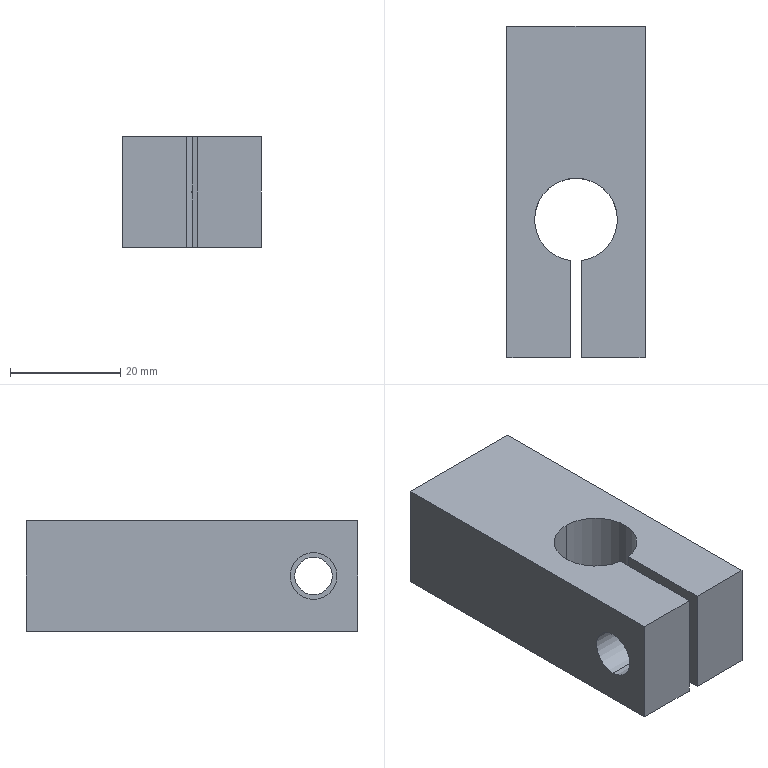Component | SolidWorks | KSD171005A-01-01-20-1 | 1 solid | 19 faces | box 25 x 60 x 20 mm | volume 21844 mm3 | plane 9 | cylinder 8 | cone 2 | commonest cylinder face diameters 8.5 x2 6.8 x2 12 x2 15 x2
build123d program:
from build123d import *

# Parameters (mm, degrees)
SKETCH1_W                      = 70
SKETCH1_H                      = 25
BOSS_EXTRUDE1_DEPTH            = 20
SKETCH2_R                      = 7.5
CUT_EXTRUDE1_DEPTH             = 43.205
CUT_EXTRUDE2_DEPTH             = 43.205
M12_TAPPED_HOLE1_D             = 12
M12_TAPPED_HOLE1_DEPTH         = 24
M12_TAPPED_HOLE1_TIP           = 3.605
M8_TAPPED_HOLE1_D              = 6.8
F_8_5_8_5_DIAMETER_HOLE1_D     = 8.5
F_8_5_8_5_DIAMETER_HOLE1_DEPTH = 12
F_8_5_8_5_DIAMETER_HOLE1_TIP   = 2.554
SKETCH15_W                     = 10
SKETCH15_H                     = 25
CUT_EXTRUDE3_DEPTH             = 43.205


with BuildPart() as part:
    # Sketch1 → Boss-Extrude1 (new body)
    with BuildSketch(Plane.XY):
        Rectangle(SKETCH1_W, SKETCH1_H)
    extrude(amount=BOSS_EXTRUDE1_DEPTH)

    # Sketch2 → Cut-Extrude1 (cut, through all)
    with BuildSketch(Plane.XY.offset(20)):
        Circle(SKETCH2_R)
    extrude(amount=-CUT_EXTRUDE1_DEPTH, mode=Mode.SUBTRACT)

    # Sketch3 → Cut-Extrude2 (cut, through all)
    with BuildSketch(Plane.XY.offset(20)):
        Polygon((-40, 0), (-40, 1), (-4.904, 1), (-4.904, -1), (-40, -1), align=None)
    extrude(amount=-CUT_EXTRUDE2_DEPTH, mode=Mode.SUBTRACT)

    # M12 Tapped Hole1
    with Locations(Plane(origin=(35, 0, 0), x_dir=(0, 0, -1), z_dir=(1, 0, 0))):
        with Locations((-10, 0)):
            Hole(M12_TAPPED_HOLE1_D / 2, depth=M12_TAPPED_HOLE1_DEPTH)
            with Locations((0, 0, -(M12_TAPPED_HOLE1_DEPTH + M12_TAPPED_HOLE1_TIP / 2))):  # 118° drill point
                Cone(0, M12_TAPPED_HOLE1_D / 2, M12_TAPPED_HOLE1_TIP, mode=Mode.SUBTRACT)

    # M8 Tapped Hole1 (through all)
    with Locations(Plane(origin=(0, 12.5, 0), x_dir=(1, 0, 0), z_dir=(0, 1, 0))):
        with Locations((-17, -10)):
            Hole(M8_TAPPED_HOLE1_D / 2)

    # 8.5 _8.5_ Diameter Hole1
    with Locations(Plane(origin=(0, 12.5, 0), x_dir=(1, 0, 0), z_dir=(0, 1, 0))):
        with Locations((-17, -10)):
            Hole(F_8_5_8_5_DIAMETER_HOLE1_D / 2, depth=F_8_5_8_5_DIAMETER_HOLE1_DEPTH)
            with Locations((0, 0, -(F_8_5_8_5_DIAMETER_HOLE1_DEPTH + F_8_5_8_5_DIAMETER_HOLE1_TIP / 2))):  # 118° drill point
                Cone(0, F_8_5_8_5_DIAMETER_HOLE1_D / 2, F_8_5_8_5_DIAMETER_HOLE1_TIP, mode=Mode.SUBTRACT)

    # Sketch15 → Cut-Extrude3 (cut, through all)
    with BuildSketch(Plane.XY.offset(20)):
        with Locations((-30, 0)):
            Rectangle(SKETCH15_W, SKETCH15_H)
    extrude(amount=-CUT_EXTRUDE3_DEPTH, mode=Mode.SUBTRACT)


solid = part.part

# Placed as in the assembly
solid = solid.moved(Location((-7.111, 15.73, 397), (0, 0, 90)))
STEP:
#1=CARTESIAN_POINT('',(-0.3193,-0.05001,15.856));
#2=VERTEX_POINT('',#1);
#3=CARTESIAN_POINT('',(-0.3193,-0.05001,16.191));
#4=VERTEX_POINT('',#3);
#5=CARTESIAN_POINT('',(-0.3193,-0.05001,16.024));
#6=DIRECTION('',(-1.,-0.,0.));
#7=DIRECTION('',(0.,0.,1.));
#8=AXIS2_PLACEMENT_3D('',#5,#6,#7);
#9=CIRCLE('',#8,0.1673);
#10=EDGE_CURVE('',#2,#4,#9,.T.);
#11=ORIENTED_EDGE('',*,*,#10,.F.);
#12=CARTESIAN_POINT('',(-0.7721,-0.05001,15.856));
#13=VERTEX_POINT('',#12);
#14=CARTESIAN_POINT('',(-0.7721,-0.05001,15.856));
#15=DIRECTION('',(-1.,-0.,0.));
#16=VECTOR('',#15,39.37);
#17=LINE('',#14,#16);
#18=EDGE_CURVE('',#2,#13,#17,.T.);
#19=ORIENTED_EDGE('',*,*,#18,.T.);
#20=CARTESIAN_POINT('',(-0.7721,-0.05001,16.191));
#21=VERTEX_POINT('',#20);
#22=CARTESIAN_POINT('',(-0.7721,-0.05001,16.024));
#23=DIRECTION('',(-1.,-0.,0.));
#24=DIRECTION('',(0.,0.,1.));
#25=AXIS2_PLACEMENT_3D('',#22,#23,#24);
#26=CIRCLE('',#25,0.1673);
#27=EDGE_CURVE('',#13,#21,#26,.T.);
#28=ORIENTED_EDGE('',*,*,#27,.T.);
#29=CARTESIAN_POINT('',(-0.7721,-0.05001,16.191));
#30=DIRECTION('',(-1.,-0.,0.));
#31=VECTOR('',#30,39.37);
#32=LINE('',#29,#31);
#33=EDGE_CURVE('',#4,#21,#32,.T.);
#34=ORIENTED_EDGE('',*,*,#33,.F.);
#35=EDGE_LOOP('',(#11,#19,#28,#34));
#36=FACE_OUTER_BOUND('',#35,.T.);
#37=CARTESIAN_POINT('',(-0.7721,-0.05001,16.024));
#38=DIRECTION('',(-1.,-0.,0.));
#39=DIRECTION('',(0.,0.,1.));
#40=AXIS2_PLACEMENT_3D('',#37,#38,#39);
#41=CYLINDRICAL_SURFACE('',#40,0.1673);
#42=ADVANCED_FACE('',(#36),#41,.F.);
#43=CARTESIAN_POINT('',(0.2122,-0.05001,15.89));
#44=VERTEX_POINT('',#43);
#45=CARTESIAN_POINT('',(0.2122,-0.05001,16.157));
#46=VERTEX_POINT('',#45);
#47=CARTESIAN_POINT('',(0.2122,-0.05001,16.024));
#48=DIRECTION('',(-1.,-0.,0.));
#49=DIRECTION('',(0.,0.,1.));
#50=AXIS2_PLACEMENT_3D('',#47,#48,#49);
#51=CIRCLE('',#50,0.1339);
#52=EDGE_CURVE('',#44,#46,#51,.T.);
#53=ORIENTED_EDGE('',*,*,#52,.F.);
#54=CARTESIAN_POINT('',(-0.2406,-0.05001,15.89));
#55=VERTEX_POINT('',#54);
#56=CARTESIAN_POINT('',(-0.7721,-0.05001,15.89));
#57=DIRECTION('',(-1.,-0.,0.));
#58=VECTOR('',#57,39.37);
#59=LINE('',#56,#58);
#60=EDGE_CURVE('',#44,#55,#59,.T.);
#61=ORIENTED_EDGE('',*,*,#60,.T.);
#62=CARTESIAN_POINT('',(-0.2406,-0.05001,16.157));
#63=VERTEX_POINT('',#62);
#64=CARTESIAN_POINT('',(-0.2406,-0.05001,16.024));
#65=DIRECTION('',(1.,0.,0.));
#66=DIRECTION('',(-0.,1.,0.));
#67=AXIS2_PLACEMENT_3D('',#64,#65,#66);
#68=CIRCLE('',#67,0.1339);
#69=EDGE_CURVE('',#63,#55,#68,.T.);
#70=ORIENTED_EDGE('',*,*,#69,.F.);
#71=CARTESIAN_POINT('',(-0.7721,-0.05001,16.157));
#72=DIRECTION('',(-1.,-0.,0.));
#73=VECTOR('',#72,39.37);
#74=LINE('',#71,#73);
#75=EDGE_CURVE('',#46,#63,#74,.T.);
#76=ORIENTED_EDGE('',*,*,#75,.F.);
#77=EDGE_LOOP('',(#53,#61,#70,#76));
#78=FACE_OUTER_BOUND('',#77,.T.);
#79=CARTESIAN_POINT('',(-0.7721,-0.05001,16.024));
#80=DIRECTION('',(-1.,-0.,0.));
#81=DIRECTION('',(0.,0.,1.));
#82=AXIS2_PLACEMENT_3D('',#79,#80,#81);
#83=CYLINDRICAL_SURFACE('',#82,0.1339);
#84=ADVANCED_FACE('',(#78),#83,.F.);
#85=CARTESIAN_POINT('',(-0.28,1.052,16.26));
#86=VERTEX_POINT('',#85);
#87=CARTESIAN_POINT('',(-0.28,1.052,15.787));
#88=VERTEX_POINT('',#87);
#89=CARTESIAN_POINT('',(-0.28,1.052,16.024));
#90=DIRECTION('',(-0.,1.,0.));
#91=DIRECTION('',(0.,0.,-1.));
#92=AXIS2_PLACEMENT_3D('',#89,#90,#91);
#93=CIRCLE('',#92,0.2362);
#94=EDGE_CURVE('',#86,#88,#93,.T.);
#95=ORIENTED_EDGE('',*,*,#94,.F.);
#96=CARTESIAN_POINT('',(-0.28,1.997,16.26));
#97=VERTEX_POINT('',#96);
#98=CARTESIAN_POINT('',(-0.28,1.997,16.26));
#99=DIRECTION('',(-0.,1.,0.));
#100=VECTOR('',#99,39.37);
#101=LINE('',#98,#100);
#102=EDGE_CURVE('',#86,#97,#101,.T.);
#103=ORIENTED_EDGE('',*,*,#102,.T.);
#104=CARTESIAN_POINT('',(-0.28,1.997,15.787));
#105=VERTEX_POINT('',#104);
#106=CARTESIAN_POINT('',(-0.28,1.997,16.024));
#107=DIRECTION('',(-0.,1.,0.));
#108=DIRECTION('',(0.,0.,-1.));
#109=AXIS2_PLACEMENT_3D('',#106,#107,#108);
#110=CIRCLE('',#109,0.2362);
#111=EDGE_CURVE('',#97,#105,#110,.T.);
#112=ORIENTED_EDGE('',*,*,#111,.T.);
#113=CARTESIAN_POINT('',(-0.28,1.997,15.787));
#114=DIRECTION('',(-0.,1.,0.));
#115=VECTOR('',#114,39.37);
#116=LINE('',#113,#115);
#117=EDGE_CURVE('',#88,#105,#116,.T.);
#118=ORIENTED_EDGE('',*,*,#117,.F.);
#119=EDGE_LOOP('',(#95,#103,#112,#118));
#120=FACE_OUTER_BOUND('',#119,.T.);
#121=CARTESIAN_POINT('',(-0.28,1.997,16.024));
#122=DIRECTION('',(-0.,1.,0.));
#123=DIRECTION('',(0.,0.,-1.));
#124=AXIS2_PLACEMENT_3D('',#121,#122,#123);
#125=CYLINDRICAL_SURFACE('',#124,0.2362);
#126=ADVANCED_FACE('',(#120),#125,.F.);
#127=CARTESIAN_POINT('',(-0.28,0.9146,16.031));
#128=VERTEX_POINT('',#127);
#129=CARTESIAN_POINT('',(-0.28,0.9146,16.017));
#130=VERTEX_POINT('',#129);
#131=CARTESIAN_POINT('',(-0.28,0.9146,16.031));
#132=CARTESIAN_POINT('',(-0.2782,0.9146,16.031));
#133=CARTESIAN_POINT('',(-0.2764,0.9145,16.03));
#134=CARTESIAN_POINT('',(-0.2739,0.9145,16.027));
#135=CARTESIAN_POINT('',(-0.2732,0.9145,16.025));
#136=CARTESIAN_POINT('',(-0.2732,0.9145,16.022));
#137=CARTESIAN_POINT('',(-0.2739,0.9145,16.02));
#138=CARTESIAN_POINT('',(-0.2764,0.9145,16.017));
#139=CARTESIAN_POINT('',(-0.2782,0.9146,16.017));
#140=CARTESIAN_POINT('',(-0.28,0.9146,16.017));
#141=B_SPLINE_CURVE_WITH_KNOTS('',3,(#131,#132,#133,#134,#135,#136,#137,#138,#139,#140),.UNSPECIFIED.,.F.,.F.,(4,2,2,2,4),(0.0006783,0.0008137,0.0009492,0.001085,0.00122),.UNSPECIFIED.);
#142=EDGE_CURVE('',#128,#130,#141,.T.);
#143=ORIENTED_EDGE('',*,*,#142,.F.);
#144=CARTESIAN_POINT('',(-0.28,1.052,16.26));
#145=DIRECTION('',(-0.,0.515,0.8572));
#146=VECTOR('',#145,39.37);
#147=LINE('',#144,#146);
#148=EDGE_CURVE('',#128,#86,#147,.T.);
#149=ORIENTED_EDGE('',*,*,#148,.T.);
#150=ORIENTED_EDGE('',*,*,#94,.T.);
#151=CARTESIAN_POINT('',(-0.28,1.052,15.787));
#152=DIRECTION('',(-0.,0.515,-0.8572));
#153=VECTOR('',#152,39.37);
#154=LINE('',#151,#153);
#155=EDGE_CURVE('',#130,#88,#154,.T.);
#156=ORIENTED_EDGE('',*,*,#155,.F.);
#157=EDGE_LOOP('',(#143,#149,#150,#156));
#158=FACE_OUTER_BOUND('',#157,.T.);
#159=CARTESIAN_POINT('',(-0.28,1.052,16.024));
#160=DIRECTION('',(-0.,1.,0.));
#161=DIRECTION('',(0.,0.,-1.));
#162=AXIS2_PLACEMENT_3D('',#159,#160,#161);
#163=CONICAL_SURFACE('',#162,0.2362,1.03);
#164=ADVANCED_FACE('',(#158),#163,.F.);
#165=CARTESIAN_POINT('',(-0.28,0.9146,15.63));
#166=VERTEX_POINT('',#165);
#167=CARTESIAN_POINT('',(-0.3193,0.3266,15.63));
#168=VERTEX_POINT('',#167);
#169=CARTESIAN_POINT('',(-0.28,0.6193,15.63));
#170=DIRECTION('',(-0.,-0.,1.));
#171=DIRECTION('',(-0.,1.,0.));
#172=AXIS2_PLACEMENT_3D('',#169,#170,#171);
#173=CIRCLE('',#172,0.2953);
#174=EDGE_CURVE('',#166,#168,#173,.T.);
#175=ORIENTED_EDGE('',*,*,#174,.F.);
#176=CARTESIAN_POINT('',(-0.28,0.9146,15.63));
#177=DIRECTION('',(-0.,-0.,1.));
#178=VECTOR('',#177,39.37);
#179=LINE('',#176,#178);
#180=EDGE_CURVE('',#166,#130,#179,.T.);
#181=ORIENTED_EDGE('',*,*,#180,.T.);
#182=CARTESIAN_POINT('',(-0.28,0.9146,16.017));
#183=CARTESIAN_POINT('',(-0.2818,0.9146,16.017));
#184=CARTESIAN_POINT('',(-0.2835,0.9145,16.017));
#185=CARTESIAN_POINT('',(-0.286,0.9145,16.02));
#186=CARTESIAN_POINT('',(-0.2867,0.9145,16.022));
#187=CARTESIAN_POINT('',(-0.2867,0.9145,16.025));
#188=CARTESIAN_POINT('',(-0.286,0.9145,16.027));
#189=CARTESIAN_POINT('',(-0.2835,0.9145,16.03));
#190=CARTESIAN_POINT('',(-0.2818,0.9146,16.031));
#191=CARTESIAN_POINT('',(-0.28,0.9146,16.031));
#192=B_SPLINE_CURVE_WITH_KNOTS('',3,(#182,#183,#184,#185,#186,#187,#188,#189,#190,#191),.UNSPECIFIED.,.F.,.F.,(4,2,2,2,4),(0.000136,0.0002716,0.0004071,0.0005427,0.0006783),.UNSPECIFIED.);
#193=EDGE_CURVE('',#130,#128,#192,.T.);
#194=ORIENTED_EDGE('',*,*,#193,.T.);
#195=CARTESIAN_POINT('',(-0.28,0.9146,16.417));
#196=VERTEX_POINT('',#195);
#197=CARTESIAN_POINT('',(-0.28,0.9146,15.63));
#198=DIRECTION('',(-0.,-0.,1.));
#199=VECTOR('',#198,39.37);
#200=LINE('',#197,#199);
#201=EDGE_CURVE('',#128,#196,#200,.T.);
#202=ORIENTED_EDGE('',*,*,#201,.T.);
#203=CARTESIAN_POINT('',(-0.3193,0.3266,16.417));
#204=VERTEX_POINT('',#203);
#205=CARTESIAN_POINT('',(-0.28,0.6193,16.417));
#206=DIRECTION('',(-0.,-0.,1.));
#207=DIRECTION('',(-0.,1.,0.));
#208=AXIS2_PLACEMENT_3D('',#205,#206,#207);
#209=CIRCLE('',#208,0.2953);
#210=EDGE_CURVE('',#196,#204,#209,.T.);
#211=ORIENTED_EDGE('',*,*,#210,.T.);
#212=CARTESIAN_POINT('',(-0.3193,0.3266,15.63));
#213=DIRECTION('',(0.,0.,-1.));
#214=VECTOR('',#213,39.37);
#215=LINE('',#212,#214);
#216=EDGE_CURVE('',#204,#168,#215,.T.);
#217=ORIENTED_EDGE('',*,*,#216,.T.);
#218=EDGE_LOOP('',(#175,#181,#194,#202,#211,#217));
#219=FACE_OUTER_BOUND('',#218,.T.);
#220=CARTESIAN_POINT('',(-0.28,0.6193,15.63));
#221=DIRECTION('',(-0.,-0.,1.));
#222=DIRECTION('',(-0.,1.,0.));
#223=AXIS2_PLACEMENT_3D('',#220,#221,#222);
#224=CYLINDRICAL_SURFACE('',#223,0.2953);
#225=ADVANCED_FACE('',(#219),#224,.F.);
#226=CARTESIAN_POINT('',(-0.28,1.997,16.024));
#227=DIRECTION('',(-0.,1.,0.));
#228=DIRECTION('',(0.,0.,-1.));
#229=AXIS2_PLACEMENT_3D('',#226,#227,#228);
#230=CIRCLE('',#229,0.2362);
#231=EDGE_CURVE('',#105,#97,#230,.T.);
#232=ORIENTED_EDGE('',*,*,#231,.F.);
#233=ORIENTED_EDGE('',*,*,#111,.F.);
#234=EDGE_LOOP('',(#232,#233));
#235=FACE_BOUND('',#234,.T.);
#236=CARTESIAN_POINT('',(0.2122,1.997,15.63));
#237=VERTEX_POINT('',#236);
#238=CARTESIAN_POINT('',(-0.7721,1.997,15.63));
#239=VERTEX_POINT('',#238);
#240=CARTESIAN_POINT('',(-0.7721,1.997,15.63));
#241=DIRECTION('',(-1.,-0.,-0.));
#242=VECTOR('',#241,39.37);
#243=LINE('',#240,#242);
#244=EDGE_CURVE('',#237,#239,#243,.T.);
#245=ORIENTED_EDGE('',*,*,#244,.T.);
#246=CARTESIAN_POINT('',(-0.7721,1.997,16.417));
#247=VERTEX_POINT('',#246);
#248=CARTESIAN_POINT('',(-0.7721,1.997,16.417));
#249=DIRECTION('',(0.,0.,-1.));
#250=VECTOR('',#249,39.37);
#251=LINE('',#248,#250);
#252=EDGE_CURVE('',#247,#239,#251,.T.);
#253=ORIENTED_EDGE('',*,*,#252,.F.);
#254=CARTESIAN_POINT('',(0.2122,1.997,16.417));
#255=VERTEX_POINT('',#254);
#256=CARTESIAN_POINT('',(-0.7721,1.997,16.417));
#257=DIRECTION('',(-1.,-0.,-0.));
#258=VECTOR('',#257,39.37);
#259=LINE('',#256,#258);
#260=EDGE_CURVE('',#255,#247,#259,.T.);
#261=ORIENTED_EDGE('',*,*,#260,.F.);
#262=CARTESIAN_POINT('',(0.2122,1.997,16.417));
#263=DIRECTION('',(0.,0.,-1.));
#264=VECTOR('',#263,39.37);
#265=LINE('',#262,#264);
#266=EDGE_CURVE('',#255,#237,#265,.T.);
#267=ORIENTED_EDGE('',*,*,#266,.T.);
#268=EDGE_LOOP('',(#245,#253,#261,#267));
#269=FACE_OUTER_BOUND('',#268,.T.);
#270=CARTESIAN_POINT('',(-0.7721,1.997,16.417));
#271=DIRECTION('',(0.,-1.,-0.));
#272=DIRECTION('',(1.,0.,0.));
#273=AXIS2_PLACEMENT_3D('',#270,#271,#272);
#274=PLANE('',#273);
#275=ADVANCED_FACE('',(#235,#269),#274,.F.);
#276=CARTESIAN_POINT('',(-0.7721,-0.05001,16.024));
#277=DIRECTION('',(-1.,-0.,0.));
#278=DIRECTION('',(0.,0.,1.));
#279=AXIS2_PLACEMENT_3D('',#276,#277,#278);
#280=CIRCLE('',#279,0.1673);
#281=EDGE_CURVE('',#21,#13,#280,.T.);
#282=ORIENTED_EDGE('',*,*,#281,.F.);
#283=ORIENTED_EDGE('',*,*,#27,.F.);
#284=EDGE_LOOP('',(#282,#283));
#285=FACE_BOUND('',#284,.T.);
#286=CARTESIAN_POINT('',(-0.7721,-0.365,15.63));
#287=VERTEX_POINT('',#286);
#288=CARTESIAN_POINT('',(-0.7721,-0.7587,15.63));
#289=DIRECTION('',(0.,-1.,-0.));
#290=VECTOR('',#289,39.37);
#291=LINE('',#288,#290);
#292=EDGE_CURVE('',#239,#287,#291,.T.);
#293=ORIENTED_EDGE('',*,*,#292,.T.);
#294=CARTESIAN_POINT('',(-0.7721,-0.365,16.417));
#295=VERTEX_POINT('',#294);
#296=CARTESIAN_POINT('',(-0.7721,-0.365,15.63));
#297=DIRECTION('',(-0.,-0.,1.));
#298=VECTOR('',#297,39.37);
#299=LINE('',#296,#298);
#300=EDGE_CURVE('',#287,#295,#299,.T.);
#301=ORIENTED_EDGE('',*,*,#300,.T.);
#302=CARTESIAN_POINT('',(-0.7721,-0.7587,16.417));
#303=DIRECTION('',(0.,-1.,-0.));
#304=VECTOR('',#303,39.37);
#305=LINE('',#302,#304);
#306=EDGE_CURVE('',#247,#295,#305,.T.);
#307=ORIENTED_EDGE('',*,*,#306,.F.);
#308=ORIENTED_EDGE('',*,*,#252,.T.);
#309=EDGE_LOOP('',(#293,#301,#307,#308));
#310=FACE_OUTER_BOUND('',#309,.T.);
#311=CARTESIAN_POINT('',(-0.7721,-0.7587,16.417));
#312=DIRECTION('',(1.,0.,0.));
#313=DIRECTION('',(0.,0.,-1.));
#314=AXIS2_PLACEMENT_3D('',#311,#312,#313);
#315=PLANE('',#314);
#316=ADVANCED_FACE('',(#285,#310),#315,.F.);
#317=CARTESIAN_POINT('',(0.2122,-0.05001,16.024));
#318=DIRECTION('',(-1.,-0.,0.));
#319=DIRECTION('',(0.,0.,1.));
#320=AXIS2_PLACEMENT_3D('',#317,#318,#319);
#321=CIRCLE('',#320,0.1339);
#322=EDGE_CURVE('',#46,#44,#321,.T.);
#323=ORIENTED_EDGE('',*,*,#322,.T.);
#324=ORIENTED_EDGE('',*,*,#52,.T.);
#325=EDGE_LOOP('',(#323,#324));
#326=FACE_BOUND('',#325,.T.);
#327=CARTESIAN_POINT('',(0.2122,-0.365,16.417));
#328=VERTEX_POINT('',#327);
#329=CARTESIAN_POINT('',(0.2122,-0.7587,16.417));
#330=DIRECTION('',(-0.,1.,0.));
#331=VECTOR('',#330,39.37);
#332=LINE('',#329,#331);
#333=EDGE_CURVE('',#328,#255,#332,.T.);
#334=ORIENTED_EDGE('',*,*,#333,.F.);
#335=CARTESIAN_POINT('',(0.2122,-0.365,15.63));
#336=VERTEX_POINT('',#335);
#337=CARTESIAN_POINT('',(0.2122,-0.365,15.63));
#338=DIRECTION('',(-0.,-0.,1.));
#339=VECTOR('',#338,39.37);
#340=LINE('',#337,#339);
#341=EDGE_CURVE('',#336,#328,#340,.T.);
#342=ORIENTED_EDGE('',*,*,#341,.F.);
#343=CARTESIAN_POINT('',(0.2122,-0.7587,15.63));
#344=DIRECTION('',(-0.,1.,0.));
#345=VECTOR('',#344,39.37);
#346=LINE('',#343,#345);
#347=EDGE_CURVE('',#336,#237,#346,.T.);
#348=ORIENTED_EDGE('',*,*,#347,.T.);
#349=ORIENTED_EDGE('',*,*,#266,.F.);
#350=EDGE_LOOP('',(#334,#342,#348,#349));
#351=FACE_OUTER_BOUND('',#350,.T.);
#352=CARTESIAN_POINT('',(0.2122,-0.7587,16.417));
#353=DIRECTION('',(-1.,-0.,-0.));
#354=DIRECTION('',(-0.,-0.,1.));
#355=AXIS2_PLACEMENT_3D('',#352,#353,#354);
#356=PLANE('',#355);
#357=ADVANCED_FACE('',(#326,#351),#356,.F.);
#358=CARTESIAN_POINT('',(-0.2406,-0.365,16.417));
#359=VERTEX_POINT('',#358);
#360=CARTESIAN_POINT('',(-0.7721,-0.365,16.417));
#361=DIRECTION('',(-1.,-0.,0.));
#362=VECTOR('',#361,39.37);
#363=LINE('',#360,#362);
#364=EDGE_CURVE('',#328,#359,#363,.T.);
#365=ORIENTED_EDGE('',*,*,#364,.F.);
#366=ORIENTED_EDGE('',*,*,#333,.T.);
#367=ORIENTED_EDGE('',*,*,#260,.T.);
#368=ORIENTED_EDGE('',*,*,#306,.T.);
#369=CARTESIAN_POINT('',(-0.3193,-0.365,16.417));
#370=VERTEX_POINT('',#369);
#371=CARTESIAN_POINT('',(-0.7721,-0.365,16.417));
#372=DIRECTION('',(-1.,-0.,0.));
#373=VECTOR('',#372,39.37);
#374=LINE('',#371,#373);
#375=EDGE_CURVE('',#370,#295,#374,.T.);
#376=ORIENTED_EDGE('',*,*,#375,.F.);
#377=CARTESIAN_POINT('',(-0.3193,-0.9555,16.417));
#378=DIRECTION('',(0.,-1.,-0.));
#379=VECTOR('',#378,39.37);
#380=LINE('',#377,#379);
#381=EDGE_CURVE('',#204,#370,#380,.T.);
#382=ORIENTED_EDGE('',*,*,#381,.F.);
#383=ORIENTED_EDGE('',*,*,#210,.F.);
#384=CARTESIAN_POINT('',(-0.2406,0.3266,16.417));
#385=VERTEX_POINT('',#384);
#386=CARTESIAN_POINT('',(-0.28,0.6193,16.417));
#387=DIRECTION('',(-0.,-0.,1.));
#388=DIRECTION('',(-0.,1.,0.));
#389=AXIS2_PLACEMENT_3D('',#386,#387,#388);
#390=CIRCLE('',#389,0.2953);
#391=EDGE_CURVE('',#385,#196,#390,.T.);
#392=ORIENTED_EDGE('',*,*,#391,.F.);
#393=CARTESIAN_POINT('',(-0.2406,0.4262,16.417));
#394=DIRECTION('',(-0.,1.,0.));
#395=VECTOR('',#394,39.37);
#396=LINE('',#393,#395);
#397=EDGE_CURVE('',#359,#385,#396,.T.);
#398=ORIENTED_EDGE('',*,*,#397,.F.);
#399=EDGE_LOOP('',(#365,#366,#367,#368,#376,#382,#383,#392,#398));
#400=FACE_OUTER_BOUND('',#399,.T.);
#401=CARTESIAN_POINT('',(-0.28,0.6193,16.417));
#402=DIRECTION('',(-0.,-0.,1.));
#403=DIRECTION('',(-0.,1.,0.));
#404=AXIS2_PLACEMENT_3D('',#401,#402,#403);
#405=PLANE('',#404);
#406=ADVANCED_FACE('',(#400),#405,.T.);
#407=ORIENTED_EDGE('',*,*,#347,.F.);
#408=CARTESIAN_POINT('',(-0.2406,-0.365,15.63));
#409=VERTEX_POINT('',#408);
#410=CARTESIAN_POINT('',(-0.7721,-0.365,15.63));
#411=DIRECTION('',(-1.,-0.,0.));
#412=VECTOR('',#411,39.37);
#413=LINE('',#410,#412);
#414=EDGE_CURVE('',#336,#409,#413,.T.);
#415=ORIENTED_EDGE('',*,*,#414,.T.);
#416=CARTESIAN_POINT('',(-0.2406,0.3266,15.63));
#417=VERTEX_POINT('',#416);
#418=CARTESIAN_POINT('',(-0.2406,0.4262,15.63));
#419=DIRECTION('',(-0.,1.,0.));
#420=VECTOR('',#419,39.37);
#421=LINE('',#418,#420);
#422=EDGE_CURVE('',#409,#417,#421,.T.);
#423=ORIENTED_EDGE('',*,*,#422,.T.);
#424=CARTESIAN_POINT('',(-0.28,0.6193,15.63));
#425=DIRECTION('',(-0.,-0.,1.));
#426=DIRECTION('',(-0.,1.,0.));
#427=AXIS2_PLACEMENT_3D('',#424,#425,#426);
#428=CIRCLE('',#427,0.2953);
#429=EDGE_CURVE('',#417,#166,#428,.T.);
#430=ORIENTED_EDGE('',*,*,#429,.T.);
#431=ORIENTED_EDGE('',*,*,#174,.T.);
#432=CARTESIAN_POINT('',(-0.3193,-0.365,15.63));
#433=VERTEX_POINT('',#432);
#434=CARTESIAN_POINT('',(-0.3193,-0.9555,15.63));
#435=DIRECTION('',(0.,-1.,-0.));
#436=VECTOR('',#435,39.37);
#437=LINE('',#434,#436);
#438=EDGE_CURVE('',#168,#433,#437,.T.);
#439=ORIENTED_EDGE('',*,*,#438,.T.);
#440=CARTESIAN_POINT('',(-0.7721,-0.365,15.63));
#441=DIRECTION('',(-1.,-0.,0.));
#442=VECTOR('',#441,39.37);
#443=LINE('',#440,#442);
#444=EDGE_CURVE('',#433,#287,#443,.T.);
#445=ORIENTED_EDGE('',*,*,#444,.T.);
#446=ORIENTED_EDGE('',*,*,#292,.F.);
#447=ORIENTED_EDGE('',*,*,#244,.F.);
#448=EDGE_LOOP('',(#407,#415,#423,#430,#431,#439,#445,#446,#447));
#449=FACE_OUTER_BOUND('',#448,.T.);
#450=CARTESIAN_POINT('',(-0.28,0.6193,15.63));
#451=DIRECTION('',(-0.,-0.,1.));
#452=DIRECTION('',(-0.,1.,0.));
#453=AXIS2_PLACEMENT_3D('',#450,#451,#452);
#454=PLANE('',#453);
#455=ADVANCED_FACE('',(#449),#454,.F.);
#456=ORIENTED_EDGE('',*,*,#180,.F.);
#457=ORIENTED_EDGE('',*,*,#429,.F.);
#458=CARTESIAN_POINT('',(-0.2406,0.3266,15.63));
#459=DIRECTION('',(-0.,-0.,1.));
#460=VECTOR('',#459,39.37);
#461=LINE('',#458,#460);
#462=EDGE_CURVE('',#417,#385,#461,.T.);
#463=ORIENTED_EDGE('',*,*,#462,.T.);
#464=ORIENTED_EDGE('',*,*,#391,.T.);
#465=ORIENTED_EDGE('',*,*,#201,.F.);
#466=ORIENTED_EDGE('',*,*,#142,.T.);
#467=EDGE_LOOP('',(#456,#457,#463,#464,#465,#466));
#468=FACE_OUTER_BOUND('',#467,.T.);
#469=CARTESIAN_POINT('',(-0.28,0.6193,15.63));
#470=DIRECTION('',(-0.,-0.,1.));
#471=DIRECTION('',(-0.,1.,0.));
#472=AXIS2_PLACEMENT_3D('',#469,#470,#471);
#473=CYLINDRICAL_SURFACE('',#472,0.2953);
#474=ADVANCED_FACE('',(#468),#473,.F.);
#475=ORIENTED_EDGE('',*,*,#69,.T.);
#476=CARTESIAN_POINT('',(-0.2406,-0.05001,16.024));
#477=DIRECTION('',(1.,0.,0.));
#478=DIRECTION('',(-0.,1.,0.));
#479=AXIS2_PLACEMENT_3D('',#476,#477,#478);
#480=CIRCLE('',#479,0.1339);
#481=EDGE_CURVE('',#55,#63,#480,.T.);
#482=ORIENTED_EDGE('',*,*,#481,.T.);
#483=EDGE_LOOP('',(#475,#482));
#484=FACE_BOUND('',#483,.T.);
#485=ORIENTED_EDGE('',*,*,#422,.F.);
#486=CARTESIAN_POINT('',(-0.2406,-0.365,15.63));
#487=DIRECTION('',(-0.,-0.,1.));
#488=VECTOR('',#487,39.37);
#489=LINE('',#486,#488);
#490=EDGE_CURVE('',#409,#359,#489,.T.);
#491=ORIENTED_EDGE('',*,*,#490,.T.);
#492=ORIENTED_EDGE('',*,*,#397,.T.);
#493=ORIENTED_EDGE('',*,*,#462,.F.);
#494=EDGE_LOOP('',(#485,#491,#492,#493));
#495=FACE_OUTER_BOUND('',#494,.T.);
#496=CARTESIAN_POINT('',(-0.2406,0.4262,15.63));
#497=DIRECTION('',(1.,0.,0.));
#498=DIRECTION('',(-0.,1.,0.));
#499=AXIS2_PLACEMENT_3D('',#496,#497,#498);
#500=PLANE('',#499);
#501=ADVANCED_FACE('',(#484,#495),#500,.F.);
#502=CARTESIAN_POINT('',(-0.3193,-0.05001,16.024));
#503=DIRECTION('',(-1.,-0.,0.));
#504=DIRECTION('',(0.,0.,1.));
#505=AXIS2_PLACEMENT_3D('',#502,#503,#504);
#506=CIRCLE('',#505,0.1673);
#507=EDGE_CURVE('',#4,#2,#506,.T.);
#508=ORIENTED_EDGE('',*,*,#507,.T.);
#509=ORIENTED_EDGE('',*,*,#10,.T.);
#510=EDGE_LOOP('',(#508,#509));
#511=FACE_BOUND('',#510,.T.);
#512=ORIENTED_EDGE('',*,*,#381,.T.);
#513=CARTESIAN_POINT('',(-0.3193,-0.365,15.63));
#514=DIRECTION('',(0.,0.,-1.));
#515=VECTOR('',#514,39.37);
#516=LINE('',#513,#515);
#517=EDGE_CURVE('',#370,#433,#516,.T.);
#518=ORIENTED_EDGE('',*,*,#517,.T.);
#519=ORIENTED_EDGE('',*,*,#438,.F.);
#520=ORIENTED_EDGE('',*,*,#216,.F.);
#521=EDGE_LOOP('',(#512,#518,#519,#520));
#522=FACE_OUTER_BOUND('',#521,.T.);
#523=CARTESIAN_POINT('',(-0.3193,-0.9555,15.63));
#524=DIRECTION('',(-1.,-0.,-0.));
#525=DIRECTION('',(-0.,-0.,1.));
#526=AXIS2_PLACEMENT_3D('',#523,#524,#525);
#527=PLANE('',#526);
#528=ADVANCED_FACE('',(#511,#522),#527,.F.);
#529=ORIENTED_EDGE('',*,*,#148,.F.);
#530=ORIENTED_EDGE('',*,*,#193,.F.);
#531=ORIENTED_EDGE('',*,*,#155,.T.);
#532=CARTESIAN_POINT('',(-0.28,1.052,16.024));
#533=DIRECTION('',(-0.,1.,0.));
#534=DIRECTION('',(0.,0.,-1.));
#535=AXIS2_PLACEMENT_3D('',#532,#533,#534);
#536=CIRCLE('',#535,0.2362);
#537=EDGE_CURVE('',#88,#86,#536,.T.);
#538=ORIENTED_EDGE('',*,*,#537,.T.);
#539=EDGE_LOOP('',(#529,#530,#531,#538));
#540=FACE_OUTER_BOUND('',#539,.T.);
#541=CARTESIAN_POINT('',(-0.28,1.052,16.024));
#542=DIRECTION('',(-0.,1.,0.));
#543=DIRECTION('',(0.,0.,-1.));
#544=AXIS2_PLACEMENT_3D('',#541,#542,#543);
#545=CONICAL_SURFACE('',#544,0.2362,1.03);
#546=ADVANCED_FACE('',(#540),#545,.F.);
#547=ORIENTED_EDGE('',*,*,#102,.F.);
#548=ORIENTED_EDGE('',*,*,#537,.F.);
#549=ORIENTED_EDGE('',*,*,#117,.T.);
#550=ORIENTED_EDGE('',*,*,#231,.T.);
#551=EDGE_LOOP('',(#547,#548,#549,#550));
#552=FACE_OUTER_BOUND('',#551,.T.);
#553=CARTESIAN_POINT('',(-0.28,1.997,16.024));
#554=DIRECTION('',(-0.,1.,0.));
#555=DIRECTION('',(0.,0.,-1.));
#556=AXIS2_PLACEMENT_3D('',#553,#554,#555);
#557=CYLINDRICAL_SURFACE('',#556,0.2362);
#558=ADVANCED_FACE('',(#552),#557,.F.);
#559=ORIENTED_EDGE('',*,*,#60,.F.);
#560=ORIENTED_EDGE('',*,*,#322,.F.);
#561=ORIENTED_EDGE('',*,*,#75,.T.);
#562=ORIENTED_EDGE('',*,*,#481,.F.);
#563=EDGE_LOOP('',(#559,#560,#561,#562));
#564=FACE_OUTER_BOUND('',#563,.T.);
#565=CARTESIAN_POINT('',(-0.7721,-0.05001,16.024));
#566=DIRECTION('',(-1.,-0.,0.));
#567=DIRECTION('',(0.,0.,1.));
#568=AXIS2_PLACEMENT_3D('',#565,#566,#567);
#569=CYLINDRICAL_SURFACE('',#568,0.1339);
#570=ADVANCED_FACE('',(#564),#569,.F.);
#571=ORIENTED_EDGE('',*,*,#18,.F.);
#572=ORIENTED_EDGE('',*,*,#507,.F.);
#573=ORIENTED_EDGE('',*,*,#33,.T.);
#574=ORIENTED_EDGE('',*,*,#281,.T.);
#575=EDGE_LOOP('',(#571,#572,#573,#574));
#576=FACE_OUTER_BOUND('',#575,.T.);
#577=CARTESIAN_POINT('',(-0.7721,-0.05001,16.024));
#578=DIRECTION('',(-1.,-0.,0.));
#579=DIRECTION('',(0.,0.,1.));
#580=AXIS2_PLACEMENT_3D('',#577,#578,#579);
#581=CYLINDRICAL_SURFACE('',#580,0.1673);
#582=ADVANCED_FACE('',(#576),#581,.F.);
#583=ORIENTED_EDGE('',*,*,#375,.T.);
#584=ORIENTED_EDGE('',*,*,#300,.F.);
#585=ORIENTED_EDGE('',*,*,#444,.F.);
#586=ORIENTED_EDGE('',*,*,#517,.F.);
#587=EDGE_LOOP('',(#583,#584,#585,#586));
#588=FACE_OUTER_BOUND('',#587,.T.);
#589=CARTESIAN_POINT('',(-0.7721,-0.365,15.63));
#590=DIRECTION('',(-0.,1.,0.));
#591=DIRECTION('',(0.,0.,-1.));
#592=AXIS2_PLACEMENT_3D('',#589,#590,#591);
#593=PLANE('',#592);
#594=ADVANCED_FACE('',(#588),#593,.F.);
#595=ORIENTED_EDGE('',*,*,#414,.F.);
#596=ORIENTED_EDGE('',*,*,#341,.T.);
#597=ORIENTED_EDGE('',*,*,#364,.T.);
#598=ORIENTED_EDGE('',*,*,#490,.F.);
#599=EDGE_LOOP('',(#595,#596,#597,#598));
#600=FACE_OUTER_BOUND('',#599,.T.);
#601=CARTESIAN_POINT('',(-0.7721,-0.365,15.63));
#602=DIRECTION('',(-0.,1.,0.));
#603=DIRECTION('',(0.,0.,-1.));
#604=AXIS2_PLACEMENT_3D('',#601,#602,#603);
#605=PLANE('',#604);
#606=ADVANCED_FACE('',(#600),#605,.F.);
#607=CLOSED_SHELL('',(#42,#84,#126,#164,#225,#275,#316,#357,#406,#455,#474,#501,#528,#546,#558,#570,#582,#594,#606));
#608=MANIFOLD_SOLID_BREP('',#607);
#609=CARTESIAN_POINT('',(0.,0.,0.));
#610=DIRECTION('',(0.,0.,1.));
#611=DIRECTION('',(1.,0.,0.));
#612=AXIS2_PLACEMENT_3D('',#609,#610,#611);
#613=(LENGTH_UNIT()NAMED_UNIT(*)SI_UNIT($,.METRE.));
#614=LENGTH_MEASURE_WITH_UNIT(LENGTH_MEASURE(0.0254),#613);
#615=DIMENSIONAL_EXPONENTS(1.,0.,0.,0.,0.,0.,0.);
#616=(CONVERSION_BASED_UNIT('',#614)LENGTH_UNIT()NAMED_UNIT(#615));
#617=UNCERTAINTY_MEASURE_WITH_UNIT(LENGTH_MEASURE(0.00001),#616,'','');
#618=(NAMED_UNIT(*)PLANE_ANGLE_UNIT()SI_UNIT($,.RADIAN.));
#619=(NAMED_UNIT(*)SI_UNIT($,.STERADIAN.)SOLID_ANGLE_UNIT());
#620=(GEOMETRIC_REPRESENTATION_CONTEXT(3)GLOBAL_UNCERTAINTY_ASSIGNED_CONTEXT((#617))GLOBAL_UNIT_ASSIGNED_CONTEXT((#616,#618,#619))REPRESENTATION_CONTEXT('',''));
#621=ADVANCED_BREP_SHAPE_REPRESENTATION('',(#608,#612),#620);
#622=COLOUR_RGB('',0.7922,0.8196,0.9333);
#623=FILL_AREA_STYLE_COLOUR('',#622);
#624=FILL_AREA_STYLE('',(#623));
#625=SURFACE_STYLE_FILL_AREA(#624);
#626=SURFACE_SIDE_STYLE('',(#625));
#627=SURFACE_STYLE_USAGE(.BOTH.,#626);
#628=PRESENTATION_STYLE_ASSIGNMENT((#627));
#629=STYLED_ITEM('',(#628),#608);
#630=PRESENTATION_LAYER_ASSIGNMENT('','',(#629));
#631=(LENGTH_UNIT()NAMED_UNIT(*)SI_UNIT($,.METRE.));
#632=LENGTH_MEASURE_WITH_UNIT(LENGTH_MEASURE(0.0254),#631);
#633=DIMENSIONAL_EXPONENTS(1.,0.,0.,0.,0.,0.,0.);
#634=(CONVERSION_BASED_UNIT('',#632)LENGTH_UNIT()NAMED_UNIT(#633));
#635=UNCERTAINTY_MEASURE_WITH_UNIT(LENGTH_MEASURE(0.00001),#634,'','');
#636=(NAMED_UNIT(*)PLANE_ANGLE_UNIT()SI_UNIT($,.RADIAN.));
#637=(NAMED_UNIT(*)SI_UNIT($,.STERADIAN.)SOLID_ANGLE_UNIT());
#638=(GEOMETRIC_REPRESENTATION_CONTEXT(3)GLOBAL_UNCERTAINTY_ASSIGNED_CONTEXT((#635))GLOBAL_UNIT_ASSIGNED_CONTEXT((#634,#636,#637))REPRESENTATION_CONTEXT('',''));
#639=MECHANICAL_DESIGN_GEOMETRIC_PRESENTATION_REPRESENTATION('',(#629),#638);